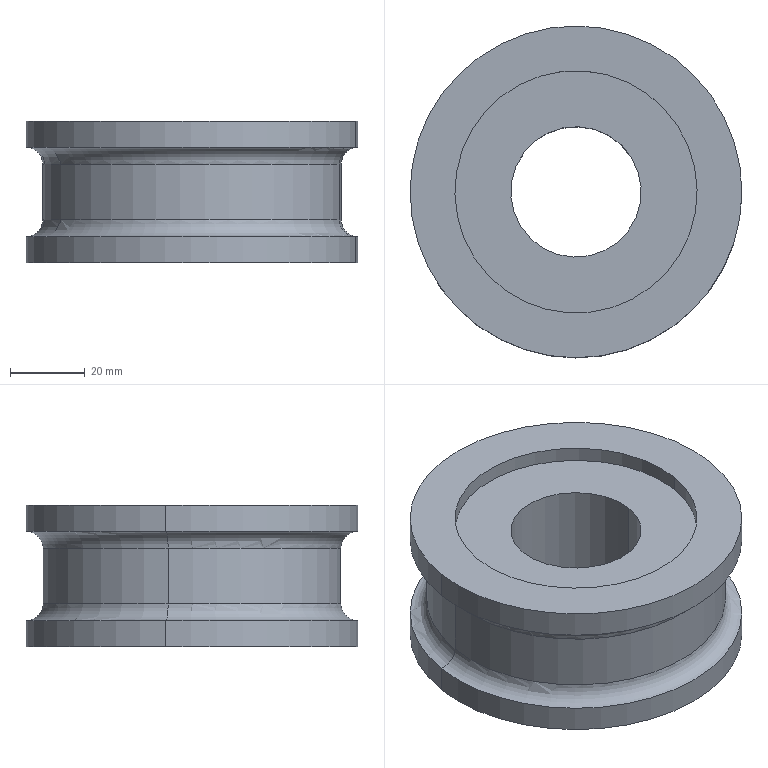Component | SolidWorks | 12AFixedFlatGrooveLargeWheel-EngravingAndMillingAxis-2_12AFlatSlotLargeStraighteningWheel-1 | 1 solid | 20 faces | box 89 x 89 x 38 mm | volume 154563 mm3 | cylinder 12 | torus 4 | plane 4 | commonest cylinder face diameters 65 x4 89 x4 35 x2 80 x2 | material GCr15
build123d program:
from build123d import *


with BuildPart() as part:
    # Sketch1 → Revolve1 (revolve)
    with BuildSketch(Plane.XY, mode=Mode.PRIVATE) as revolve1_sk:
        with BuildLine():
            Line((0, 32.5), (0, 44.5))
            Line((0, 44.5), (7, 44.5))
            ThreePointArc((7, 44.5), (8.318, 41.318), (11.5, 40))
            Line((11.5, 40), (26.5, 40))
            ThreePointArc((26.5, 40), (29.682, 41.318), (31, 44.5))
            Line((31, 44.5), (38, 44.5))
            Line((38, 44.5), (38, 32.5))
            Line((38, 32.5), (34, 32.5))
            Line((34, 32.5), (34, 17.5))
            Line((34, 17.5), (4, 17.5))
            Line((4, 17.5), (4, 32.5))
            Line((4, 32.5), (0, 32.5))
        make_face()
    revolve(revolve1_sk.sketch.rotate(Axis((0, 0, 0), (1, 0, 0)), 180), axis=Axis((0, 0, 0), (1, 0, 0)))


solid = part.part

# Placed as in the assembly
solid = solid.moved(Location((-257.402, 59.038, 55.75), (0, 90, 0)))
STEP:
#1=COLOUR_RGB('',0.7922,0.8196,0.9333);
#2=FILL_AREA_STYLE_COLOUR('',#1);
#3=FILL_AREA_STYLE('',(#2));
#4=SURFACE_STYLE_FILL_AREA(#3);
#5=SURFACE_SIDE_STYLE('',(#4));
#6=SURFACE_STYLE_USAGE(.BOTH.,#5);
#7=PRESENTATION_STYLE_ASSIGNMENT((#6));
#8=CARTESIAN_POINT('',(-9.454,2.214,0.8563));
#9=VERTEX_POINT('',#8);
#10=CARTESIAN_POINT('',(-10.814,2.435,0.8563));
#11=VERTEX_POINT('',#10);
#12=CARTESIAN_POINT('',(-10.134,2.324,0.8563));
#13=DIRECTION('',(0.,-0.,1.));
#14=DIRECTION('',(-0.9871,0.1604,0.));
#15=AXIS2_PLACEMENT_3D('',#12,#13,#14);
#16=CIRCLE('',#15,0.689);
#17=EDGE_CURVE('',#9,#11,#16,.T.);
#18=ORIENTED_EDGE('',*,*,#17,.F.);
#19=CARTESIAN_POINT('',(-9.454,2.214,2.037));
#20=VERTEX_POINT('',#19);
#21=CARTESIAN_POINT('',(-9.454,2.214,2.195));
#22=DIRECTION('',(0.,-0.,1.));
#23=VECTOR('',#22,39.37);
#24=LINE('',#21,#23);
#25=EDGE_CURVE('',#9,#20,#24,.T.);
#26=ORIENTED_EDGE('',*,*,#25,.T.);
#27=CARTESIAN_POINT('',(-10.814,2.435,2.037));
#28=VERTEX_POINT('',#27);
#29=CARTESIAN_POINT('',(-10.134,2.324,2.037));
#30=DIRECTION('',(0.,-0.,1.));
#31=DIRECTION('',(-0.9871,0.1604,0.));
#32=AXIS2_PLACEMENT_3D('',#29,#30,#31);
#33=CIRCLE('',#32,0.689);
#34=EDGE_CURVE('',#20,#28,#33,.T.);
#35=ORIENTED_EDGE('',*,*,#34,.T.);
#36=CARTESIAN_POINT('',(-10.814,2.435,2.195));
#37=DIRECTION('',(0.,-0.,1.));
#38=VECTOR('',#37,39.37);
#39=LINE('',#36,#38);
#40=EDGE_CURVE('',#11,#28,#39,.T.);
#41=ORIENTED_EDGE('',*,*,#40,.F.);
#42=EDGE_LOOP('',(#18,#26,#35,#41));
#43=FACE_OUTER_BOUND('',#42,.T.);
#44=CARTESIAN_POINT('',(-10.134,2.324,2.195));
#45=DIRECTION('',(0.,-0.,1.));
#46=DIRECTION('',(-0.9871,0.1604,0.));
#47=AXIS2_PLACEMENT_3D('',#44,#45,#46);
#48=CYLINDRICAL_SURFACE('',#47,0.689);
#49=ADVANCED_FACE('',(#43),#48,.F.);
#50=CARTESIAN_POINT('',(-8.871,2.119,2.037));
#51=VERTEX_POINT('',#50);
#52=CARTESIAN_POINT('',(-11.397,2.53,2.037));
#53=VERTEX_POINT('',#52);
#54=CARTESIAN_POINT('',(-10.134,2.324,2.037));
#55=DIRECTION('',(0.,-0.,1.));
#56=DIRECTION('',(-0.9871,0.1604,0.));
#57=AXIS2_PLACEMENT_3D('',#54,#55,#56);
#58=CIRCLE('',#57,1.28);
#59=EDGE_CURVE('',#51,#53,#58,.T.);
#60=ORIENTED_EDGE('',*,*,#59,.F.);
#61=CARTESIAN_POINT('',(-8.871,2.119,2.195));
#62=VERTEX_POINT('',#61);
#63=CARTESIAN_POINT('',(-8.871,2.119,2.195));
#64=DIRECTION('',(0.,-0.,1.));
#65=VECTOR('',#64,39.37);
#66=LINE('',#63,#65);
#67=EDGE_CURVE('',#51,#62,#66,.T.);
#68=ORIENTED_EDGE('',*,*,#67,.T.);
#69=CARTESIAN_POINT('',(-11.397,2.53,2.195));
#70=VERTEX_POINT('',#69);
#71=CARTESIAN_POINT('',(-10.134,2.324,2.195));
#72=DIRECTION('',(0.,-0.,1.));
#73=DIRECTION('',(-0.9871,0.1604,0.));
#74=AXIS2_PLACEMENT_3D('',#71,#72,#73);
#75=CIRCLE('',#74,1.28);
#76=EDGE_CURVE('',#62,#70,#75,.T.);
#77=ORIENTED_EDGE('',*,*,#76,.T.);
#78=CARTESIAN_POINT('',(-11.397,2.53,2.195));
#79=DIRECTION('',(0.,-0.,1.));
#80=VECTOR('',#79,39.37);
#81=LINE('',#78,#80);
#82=EDGE_CURVE('',#53,#70,#81,.T.);
#83=ORIENTED_EDGE('',*,*,#82,.F.);
#84=EDGE_LOOP('',(#60,#68,#77,#83));
#85=FACE_OUTER_BOUND('',#84,.T.);
#86=CARTESIAN_POINT('',(-10.134,2.324,2.195));
#87=DIRECTION('',(0.,-0.,1.));
#88=DIRECTION('',(-0.9871,0.1604,0.));
#89=AXIS2_PLACEMENT_3D('',#86,#87,#88);
#90=CYLINDRICAL_SURFACE('',#89,1.28);
#91=ADVANCED_FACE('',(#85),#90,.F.);
#92=CARTESIAN_POINT('',(-11.863,2.605,1.919));
#93=VERTEX_POINT('',#92);
#94=CARTESIAN_POINT('',(-8.405,2.043,1.919));
#95=VERTEX_POINT('',#94);
#96=CARTESIAN_POINT('',(-10.134,2.324,1.919));
#97=DIRECTION('',(0.,-0.,1.));
#98=DIRECTION('',(-0.9871,0.1604,0.));
#99=AXIS2_PLACEMENT_3D('',#96,#97,#98);
#100=CIRCLE('',#99,1.752);
#101=EDGE_CURVE('',#93,#95,#100,.T.);
#102=ORIENTED_EDGE('',*,*,#101,.T.);
#103=CARTESIAN_POINT('',(-8.405,2.043,2.195));
#104=VERTEX_POINT('',#103);
#105=CARTESIAN_POINT('',(-8.405,2.043,2.195));
#106=DIRECTION('',(0.,-0.,1.));
#107=VECTOR('',#106,39.37);
#108=LINE('',#105,#107);
#109=EDGE_CURVE('',#95,#104,#108,.T.);
#110=ORIENTED_EDGE('',*,*,#109,.T.);
#111=CARTESIAN_POINT('',(-11.863,2.605,2.195));
#112=VERTEX_POINT('',#111);
#113=CARTESIAN_POINT('',(-10.134,2.324,2.195));
#114=DIRECTION('',(0.,-0.,1.));
#115=DIRECTION('',(-0.9871,0.1604,0.));
#116=AXIS2_PLACEMENT_3D('',#113,#114,#115);
#117=CIRCLE('',#116,1.752);
#118=EDGE_CURVE('',#112,#104,#117,.T.);
#119=ORIENTED_EDGE('',*,*,#118,.F.);
#120=CARTESIAN_POINT('',(-11.863,2.605,2.195));
#121=DIRECTION('',(0.,-0.,1.));
#122=VECTOR('',#121,39.37);
#123=LINE('',#120,#122);
#124=EDGE_CURVE('',#93,#112,#123,.T.);
#125=ORIENTED_EDGE('',*,*,#124,.F.);
#126=EDGE_LOOP('',(#102,#110,#119,#125));
#127=FACE_OUTER_BOUND('',#126,.T.);
#128=CARTESIAN_POINT('',(-10.134,2.324,2.195));
#129=DIRECTION('',(0.,-0.,1.));
#130=DIRECTION('',(-0.9871,0.1604,0.));
#131=AXIS2_PLACEMENT_3D('',#128,#129,#130);
#132=CYLINDRICAL_SURFACE('',#131,1.752);
#133=ADVANCED_FACE('',(#127),#132,.T.);
#134=CARTESIAN_POINT('',(-10.134,2.324,1.919));
#135=DIRECTION('',(0.,-0.,1.));
#136=DIRECTION('',(-0.9871,0.1604,0.));
#137=AXIS2_PLACEMENT_3D('',#134,#135,#136);
#138=CIRCLE('',#137,1.752);
#139=EDGE_CURVE('',#95,#93,#138,.T.);
#140=ORIENTED_EDGE('',*,*,#139,.F.);
#141=CARTESIAN_POINT('',(-8.58,2.072,1.742));
#142=VERTEX_POINT('',#141);
#143=CARTESIAN_POINT('',(-8.405,2.043,1.742));
#144=DIRECTION('',(-0.1604,-0.9871,-0.));
#145=DIRECTION('',(0.9871,-0.1604,0.));
#146=AXIS2_PLACEMENT_3D('',#143,#144,#145);
#147=CIRCLE('',#146,0.1772);
#148=EDGE_CURVE('',#95,#142,#147,.T.);
#149=ORIENTED_EDGE('',*,*,#148,.T.);
#150=CARTESIAN_POINT('',(-11.688,2.577,1.742));
#151=VERTEX_POINT('',#150);
#152=CARTESIAN_POINT('',(-10.134,2.324,1.742));
#153=DIRECTION('',(0.,-0.,1.));
#154=DIRECTION('',(-0.9871,0.1604,0.));
#155=AXIS2_PLACEMENT_3D('',#152,#153,#154);
#156=CIRCLE('',#155,1.575);
#157=EDGE_CURVE('',#142,#151,#156,.T.);
#158=ORIENTED_EDGE('',*,*,#157,.T.);
#159=CARTESIAN_POINT('',(-11.863,2.605,1.742));
#160=DIRECTION('',(0.1604,0.9871,0.));
#161=DIRECTION('',(-0.9871,0.1604,0.));
#162=AXIS2_PLACEMENT_3D('',#159,#160,#161);
#163=CIRCLE('',#162,0.1772);
#164=EDGE_CURVE('',#93,#151,#163,.T.);
#165=ORIENTED_EDGE('',*,*,#164,.F.);
#166=EDGE_LOOP('',(#140,#149,#158,#165));
#167=FACE_OUTER_BOUND('',#166,.T.);
#168=CARTESIAN_POINT('',(-10.134,2.324,1.742));
#169=DIRECTION('',(0.,-0.,1.));
#170=DIRECTION('',(-0.9871,0.1604,0.));
#171=AXIS2_PLACEMENT_3D('',#168,#169,#170);
#172=TOROIDAL_SURFACE('',#171,1.752,0.1772);
#173=ADVANCED_FACE('',(#167),#172,.F.);
#174=CARTESIAN_POINT('',(-11.688,2.577,1.152));
#175=VERTEX_POINT('',#174);
#176=CARTESIAN_POINT('',(-8.58,2.072,1.152));
#177=VERTEX_POINT('',#176);
#178=CARTESIAN_POINT('',(-10.134,2.324,1.152));
#179=DIRECTION('',(0.,-0.,1.));
#180=DIRECTION('',(-0.9871,0.1604,0.));
#181=AXIS2_PLACEMENT_3D('',#178,#179,#180);
#182=CIRCLE('',#181,1.575);
#183=EDGE_CURVE('',#175,#177,#182,.T.);
#184=ORIENTED_EDGE('',*,*,#183,.T.);
#185=CARTESIAN_POINT('',(-8.58,2.072,2.195));
#186=DIRECTION('',(0.,-0.,1.));
#187=VECTOR('',#186,39.37);
#188=LINE('',#185,#187);
#189=EDGE_CURVE('',#177,#142,#188,.T.);
#190=ORIENTED_EDGE('',*,*,#189,.T.);
#191=CARTESIAN_POINT('',(-10.134,2.324,1.742));
#192=DIRECTION('',(0.,-0.,1.));
#193=DIRECTION('',(-0.9871,0.1604,0.));
#194=AXIS2_PLACEMENT_3D('',#191,#192,#193);
#195=CIRCLE('',#194,1.575);
#196=EDGE_CURVE('',#151,#142,#195,.T.);
#197=ORIENTED_EDGE('',*,*,#196,.F.);
#198=CARTESIAN_POINT('',(-11.688,2.577,2.195));
#199=DIRECTION('',(0.,-0.,1.));
#200=VECTOR('',#199,39.37);
#201=LINE('',#198,#200);
#202=EDGE_CURVE('',#175,#151,#201,.T.);
#203=ORIENTED_EDGE('',*,*,#202,.F.);
#204=EDGE_LOOP('',(#184,#190,#197,#203));
#205=FACE_OUTER_BOUND('',#204,.T.);
#206=CARTESIAN_POINT('',(-10.134,2.324,2.195));
#207=DIRECTION('',(0.,-0.,1.));
#208=DIRECTION('',(-0.9871,0.1604,0.));
#209=AXIS2_PLACEMENT_3D('',#206,#207,#208);
#210=CYLINDRICAL_SURFACE('',#209,1.575);
#211=ADVANCED_FACE('',(#205),#210,.T.);
#212=CARTESIAN_POINT('',(-10.134,2.324,1.152));
#213=DIRECTION('',(0.,-0.,1.));
#214=DIRECTION('',(-0.9871,0.1604,0.));
#215=AXIS2_PLACEMENT_3D('',#212,#213,#214);
#216=CIRCLE('',#215,1.575);
#217=EDGE_CURVE('',#177,#175,#216,.T.);
#218=ORIENTED_EDGE('',*,*,#217,.F.);
#219=CARTESIAN_POINT('',(-8.405,2.043,0.9744));
#220=VERTEX_POINT('',#219);
#221=CARTESIAN_POINT('',(-8.405,2.043,1.152));
#222=DIRECTION('',(-0.1604,-0.9871,-0.));
#223=DIRECTION('',(0.9871,-0.1604,0.));
#224=AXIS2_PLACEMENT_3D('',#221,#222,#223);
#225=CIRCLE('',#224,0.1772);
#226=EDGE_CURVE('',#177,#220,#225,.T.);
#227=ORIENTED_EDGE('',*,*,#226,.T.);
#228=CARTESIAN_POINT('',(-11.863,2.605,0.9744));
#229=VERTEX_POINT('',#228);
#230=CARTESIAN_POINT('',(-10.134,2.324,0.9744));
#231=DIRECTION('',(0.,-0.,1.));
#232=DIRECTION('',(-0.9871,0.1604,0.));
#233=AXIS2_PLACEMENT_3D('',#230,#231,#232);
#234=CIRCLE('',#233,1.752);
#235=EDGE_CURVE('',#220,#229,#234,.T.);
#236=ORIENTED_EDGE('',*,*,#235,.T.);
#237=CARTESIAN_POINT('',(-11.863,2.605,1.152));
#238=DIRECTION('',(0.1604,0.9871,0.));
#239=DIRECTION('',(-0.9871,0.1604,0.));
#240=AXIS2_PLACEMENT_3D('',#237,#238,#239);
#241=CIRCLE('',#240,0.1772);
#242=EDGE_CURVE('',#175,#229,#241,.T.);
#243=ORIENTED_EDGE('',*,*,#242,.F.);
#244=EDGE_LOOP('',(#218,#227,#236,#243));
#245=FACE_OUTER_BOUND('',#244,.T.);
#246=CARTESIAN_POINT('',(-10.134,2.324,1.152));
#247=DIRECTION('',(0.,-0.,1.));
#248=DIRECTION('',(-0.9871,0.1604,0.));
#249=AXIS2_PLACEMENT_3D('',#246,#247,#248);
#250=TOROIDAL_SURFACE('',#249,1.752,0.1772);
#251=ADVANCED_FACE('',(#245),#250,.F.);
#252=CARTESIAN_POINT('',(-11.863,2.605,0.6988));
#253=VERTEX_POINT('',#252);
#254=CARTESIAN_POINT('',(-8.405,2.043,0.6988));
#255=VERTEX_POINT('',#254);
#256=CARTESIAN_POINT('',(-10.134,2.324,0.6988));
#257=DIRECTION('',(0.,-0.,1.));
#258=DIRECTION('',(-0.9871,0.1604,0.));
#259=AXIS2_PLACEMENT_3D('',#256,#257,#258);
#260=CIRCLE('',#259,1.752);
#261=EDGE_CURVE('',#253,#255,#260,.T.);
#262=ORIENTED_EDGE('',*,*,#261,.T.);
#263=CARTESIAN_POINT('',(-8.405,2.043,2.195));
#264=DIRECTION('',(0.,-0.,1.));
#265=VECTOR('',#264,39.37);
#266=LINE('',#263,#265);
#267=EDGE_CURVE('',#255,#220,#266,.T.);
#268=ORIENTED_EDGE('',*,*,#267,.T.);
#269=CARTESIAN_POINT('',(-10.134,2.324,0.9744));
#270=DIRECTION('',(0.,-0.,1.));
#271=DIRECTION('',(-0.9871,0.1604,0.));
#272=AXIS2_PLACEMENT_3D('',#269,#270,#271);
#273=CIRCLE('',#272,1.752);
#274=EDGE_CURVE('',#229,#220,#273,.T.);
#275=ORIENTED_EDGE('',*,*,#274,.F.);
#276=CARTESIAN_POINT('',(-11.863,2.605,2.195));
#277=DIRECTION('',(0.,-0.,1.));
#278=VECTOR('',#277,39.37);
#279=LINE('',#276,#278);
#280=EDGE_CURVE('',#253,#229,#279,.T.);
#281=ORIENTED_EDGE('',*,*,#280,.F.);
#282=EDGE_LOOP('',(#262,#268,#275,#281));
#283=FACE_OUTER_BOUND('',#282,.T.);
#284=CARTESIAN_POINT('',(-10.134,2.324,2.195));
#285=DIRECTION('',(0.,-0.,1.));
#286=DIRECTION('',(-0.9871,0.1604,0.));
#287=AXIS2_PLACEMENT_3D('',#284,#285,#286);
#288=CYLINDRICAL_SURFACE('',#287,1.752);
#289=ADVANCED_FACE('',(#283),#288,.T.);
#290=CARTESIAN_POINT('',(-8.871,2.119,0.6988));
#291=VERTEX_POINT('',#290);
#292=CARTESIAN_POINT('',(-11.397,2.53,0.6988));
#293=VERTEX_POINT('',#292);
#294=CARTESIAN_POINT('',(-10.134,2.324,0.6988));
#295=DIRECTION('',(0.,-0.,1.));
#296=DIRECTION('',(-0.9871,0.1604,0.));
#297=AXIS2_PLACEMENT_3D('',#294,#295,#296);
#298=CIRCLE('',#297,1.28);
#299=EDGE_CURVE('',#291,#293,#298,.T.);
#300=ORIENTED_EDGE('',*,*,#299,.F.);
#301=CARTESIAN_POINT('',(-8.871,2.119,0.8563));
#302=VERTEX_POINT('',#301);
#303=CARTESIAN_POINT('',(-8.871,2.119,2.195));
#304=DIRECTION('',(0.,-0.,1.));
#305=VECTOR('',#304,39.37);
#306=LINE('',#303,#305);
#307=EDGE_CURVE('',#291,#302,#306,.T.);
#308=ORIENTED_EDGE('',*,*,#307,.T.);
#309=CARTESIAN_POINT('',(-11.397,2.53,0.8563));
#310=VERTEX_POINT('',#309);
#311=CARTESIAN_POINT('',(-10.134,2.324,0.8563));
#312=DIRECTION('',(0.,-0.,1.));
#313=DIRECTION('',(-0.9871,0.1604,0.));
#314=AXIS2_PLACEMENT_3D('',#311,#312,#313);
#315=CIRCLE('',#314,1.28);
#316=EDGE_CURVE('',#302,#310,#315,.T.);
#317=ORIENTED_EDGE('',*,*,#316,.T.);
#318=CARTESIAN_POINT('',(-11.397,2.53,2.195));
#319=DIRECTION('',(0.,-0.,1.));
#320=VECTOR('',#319,39.37);
#321=LINE('',#318,#320);
#322=EDGE_CURVE('',#293,#310,#321,.T.);
#323=ORIENTED_EDGE('',*,*,#322,.F.);
#324=EDGE_LOOP('',(#300,#308,#317,#323));
#325=FACE_OUTER_BOUND('',#324,.T.);
#326=CARTESIAN_POINT('',(-10.134,2.324,2.195));
#327=DIRECTION('',(0.,-0.,1.));
#328=DIRECTION('',(-0.9871,0.1604,0.));
#329=AXIS2_PLACEMENT_3D('',#326,#327,#328);
#330=CYLINDRICAL_SURFACE('',#329,1.28);
#331=ADVANCED_FACE('',(#325),#330,.F.);
#332=ORIENTED_EDGE('',*,*,#307,.F.);
#333=CARTESIAN_POINT('',(-10.134,2.324,0.6988));
#334=DIRECTION('',(0.,-0.,1.));
#335=DIRECTION('',(-0.9871,0.1604,0.));
#336=AXIS2_PLACEMENT_3D('',#333,#334,#335);
#337=CIRCLE('',#336,1.28);
#338=EDGE_CURVE('',#293,#291,#337,.T.);
#339=ORIENTED_EDGE('',*,*,#338,.F.);
#340=ORIENTED_EDGE('',*,*,#322,.T.);
#341=CARTESIAN_POINT('',(-10.134,2.324,0.8563));
#342=DIRECTION('',(0.,-0.,1.));
#343=DIRECTION('',(-0.9871,0.1604,0.));
#344=AXIS2_PLACEMENT_3D('',#341,#342,#343);
#345=CIRCLE('',#344,1.28);
#346=EDGE_CURVE('',#310,#302,#345,.T.);
#347=ORIENTED_EDGE('',*,*,#346,.T.);
#348=EDGE_LOOP('',(#332,#339,#340,#347));
#349=FACE_OUTER_BOUND('',#348,.T.);
#350=CARTESIAN_POINT('',(-10.134,2.324,2.195));
#351=DIRECTION('',(0.,-0.,1.));
#352=DIRECTION('',(-0.9871,0.1604,0.));
#353=AXIS2_PLACEMENT_3D('',#350,#351,#352);
#354=CYLINDRICAL_SURFACE('',#353,1.28);
#355=ADVANCED_FACE('',(#349),#354,.F.);
#356=ORIENTED_EDGE('',*,*,#261,.F.);
#357=CARTESIAN_POINT('',(-10.134,2.324,0.6988));
#358=DIRECTION('',(0.,-0.,1.));
#359=DIRECTION('',(-0.9871,0.1604,0.));
#360=AXIS2_PLACEMENT_3D('',#357,#358,#359);
#361=CIRCLE('',#360,1.752);
#362=EDGE_CURVE('',#255,#253,#361,.T.);
#363=ORIENTED_EDGE('',*,*,#362,.F.);
#364=EDGE_LOOP('',(#356,#363));
#365=FACE_OUTER_BOUND('',#364,.T.);
#366=ORIENTED_EDGE('',*,*,#338,.T.);
#367=ORIENTED_EDGE('',*,*,#299,.T.);
#368=EDGE_LOOP('',(#366,#367));
#369=FACE_BOUND('',#368,.T.);
#370=CARTESIAN_POINT('',(-8.405,2.043,0.6988));
#371=DIRECTION('',(0.,-0.,1.));
#372=DIRECTION('',(-0.9871,0.1604,0.));
#373=AXIS2_PLACEMENT_3D('',#370,#371,#372);
#374=PLANE('',#373);
#375=ADVANCED_FACE('',(#365,#369),#374,.F.);
#376=ORIENTED_EDGE('',*,*,#267,.F.);
#377=ORIENTED_EDGE('',*,*,#362,.T.);
#378=ORIENTED_EDGE('',*,*,#280,.T.);
#379=ORIENTED_EDGE('',*,*,#235,.F.);
#380=EDGE_LOOP('',(#376,#377,#378,#379));
#381=FACE_OUTER_BOUND('',#380,.T.);
#382=CARTESIAN_POINT('',(-10.134,2.324,2.195));
#383=DIRECTION('',(0.,-0.,1.));
#384=DIRECTION('',(-0.9871,0.1604,0.));
#385=AXIS2_PLACEMENT_3D('',#382,#383,#384);
#386=CYLINDRICAL_SURFACE('',#385,1.752);
#387=ADVANCED_FACE('',(#381),#386,.T.);
#388=ORIENTED_EDGE('',*,*,#226,.F.);
#389=ORIENTED_EDGE('',*,*,#183,.F.);
#390=ORIENTED_EDGE('',*,*,#242,.T.);
#391=ORIENTED_EDGE('',*,*,#274,.T.);
#392=EDGE_LOOP('',(#388,#389,#390,#391));
#393=FACE_OUTER_BOUND('',#392,.T.);
#394=CARTESIAN_POINT('',(-10.134,2.324,1.152));
#395=DIRECTION('',(0.,-0.,1.));
#396=DIRECTION('',(-0.9871,0.1604,0.));
#397=AXIS2_PLACEMENT_3D('',#394,#395,#396);
#398=TOROIDAL_SURFACE('',#397,1.752,0.1772);
#399=ADVANCED_FACE('',(#393),#398,.F.);
#400=ORIENTED_EDGE('',*,*,#189,.F.);
#401=ORIENTED_EDGE('',*,*,#217,.T.);
#402=ORIENTED_EDGE('',*,*,#202,.T.);
#403=ORIENTED_EDGE('',*,*,#157,.F.);
#404=EDGE_LOOP('',(#400,#401,#402,#403));
#405=FACE_OUTER_BOUND('',#404,.T.);
#406=CARTESIAN_POINT('',(-10.134,2.324,2.195));
#407=DIRECTION('',(0.,-0.,1.));
#408=DIRECTION('',(-0.9871,0.1604,0.));
#409=AXIS2_PLACEMENT_3D('',#406,#407,#408);
#410=CYLINDRICAL_SURFACE('',#409,1.575);
#411=ADVANCED_FACE('',(#405),#410,.T.);
#412=ORIENTED_EDGE('',*,*,#148,.F.);
#413=ORIENTED_EDGE('',*,*,#101,.F.);
#414=ORIENTED_EDGE('',*,*,#164,.T.);
#415=ORIENTED_EDGE('',*,*,#196,.T.);
#416=EDGE_LOOP('',(#412,#413,#414,#415));
#417=FACE_OUTER_BOUND('',#416,.T.);
#418=CARTESIAN_POINT('',(-10.134,2.324,1.742));
#419=DIRECTION('',(0.,-0.,1.));
#420=DIRECTION('',(-0.9871,0.1604,0.));
#421=AXIS2_PLACEMENT_3D('',#418,#419,#420);
#422=TOROIDAL_SURFACE('',#421,1.752,0.1772);
#423=ADVANCED_FACE('',(#417),#422,.F.);
#424=ORIENTED_EDGE('',*,*,#109,.F.);
#425=ORIENTED_EDGE('',*,*,#139,.T.);
#426=ORIENTED_EDGE('',*,*,#124,.T.);
#427=CARTESIAN_POINT('',(-10.134,2.324,2.195));
#428=DIRECTION('',(0.,-0.,1.));
#429=DIRECTION('',(-0.9871,0.1604,0.));
#430=AXIS2_PLACEMENT_3D('',#427,#428,#429);
#431=CIRCLE('',#430,1.752);
#432=EDGE_CURVE('',#104,#112,#431,.T.);
#433=ORIENTED_EDGE('',*,*,#432,.F.);
#434=EDGE_LOOP('',(#424,#425,#426,#433));
#435=FACE_OUTER_BOUND('',#434,.T.);
#436=CARTESIAN_POINT('',(-10.134,2.324,2.195));
#437=DIRECTION('',(0.,-0.,1.));
#438=DIRECTION('',(-0.9871,0.1604,0.));
#439=AXIS2_PLACEMENT_3D('',#436,#437,#438);
#440=CYLINDRICAL_SURFACE('',#439,1.752);
#441=ADVANCED_FACE('',(#435),#440,.T.);
#442=CARTESIAN_POINT('',(-10.134,2.324,2.195));
#443=DIRECTION('',(0.,-0.,1.));
#444=DIRECTION('',(-0.9871,0.1604,0.));
#445=AXIS2_PLACEMENT_3D('',#442,#443,#444);
#446=CIRCLE('',#445,1.28);
#447=EDGE_CURVE('',#70,#62,#446,.T.);
#448=ORIENTED_EDGE('',*,*,#447,.F.);
#449=ORIENTED_EDGE('',*,*,#76,.F.);
#450=EDGE_LOOP('',(#448,#449));
#451=FACE_BOUND('',#450,.T.);
#452=ORIENTED_EDGE('',*,*,#118,.T.);
#453=ORIENTED_EDGE('',*,*,#432,.T.);
#454=EDGE_LOOP('',(#452,#453));
#455=FACE_OUTER_BOUND('',#454,.T.);
#456=CARTESIAN_POINT('',(-8.871,2.119,2.195));
#457=DIRECTION('',(-0.,0.,-1.));
#458=DIRECTION('',(0.9871,-0.1604,-0.));
#459=AXIS2_PLACEMENT_3D('',#456,#457,#458);
#460=PLANE('',#459);
#461=ADVANCED_FACE('',(#451,#455),#460,.F.);
#462=ORIENTED_EDGE('',*,*,#67,.F.);
#463=CARTESIAN_POINT('',(-10.134,2.324,2.037));
#464=DIRECTION('',(0.,-0.,1.));
#465=DIRECTION('',(-0.9871,0.1604,0.));
#466=AXIS2_PLACEMENT_3D('',#463,#464,#465);
#467=CIRCLE('',#466,1.28);
#468=EDGE_CURVE('',#53,#51,#467,.T.);
#469=ORIENTED_EDGE('',*,*,#468,.F.);
#470=ORIENTED_EDGE('',*,*,#82,.T.);
#471=ORIENTED_EDGE('',*,*,#447,.T.);
#472=EDGE_LOOP('',(#462,#469,#470,#471));
#473=FACE_OUTER_BOUND('',#472,.T.);
#474=CARTESIAN_POINT('',(-10.134,2.324,2.195));
#475=DIRECTION('',(0.,-0.,1.));
#476=DIRECTION('',(-0.9871,0.1604,0.));
#477=AXIS2_PLACEMENT_3D('',#474,#475,#476);
#478=CYLINDRICAL_SURFACE('',#477,1.28);
#479=ADVANCED_FACE('',(#473),#478,.F.);
#480=CARTESIAN_POINT('',(-10.134,2.324,2.037));
#481=DIRECTION('',(0.,-0.,1.));
#482=DIRECTION('',(-0.9871,0.1604,0.));
#483=AXIS2_PLACEMENT_3D('',#480,#481,#482);
#484=CIRCLE('',#483,0.689);
#485=EDGE_CURVE('',#28,#20,#484,.T.);
#486=ORIENTED_EDGE('',*,*,#485,.F.);
#487=ORIENTED_EDGE('',*,*,#34,.F.);
#488=EDGE_LOOP('',(#486,#487));
#489=FACE_BOUND('',#488,.T.);
#490=ORIENTED_EDGE('',*,*,#468,.T.);
#491=ORIENTED_EDGE('',*,*,#59,.T.);
#492=EDGE_LOOP('',(#490,#491));
#493=FACE_OUTER_BOUND('',#492,.T.);
#494=CARTESIAN_POINT('',(-8.871,2.119,2.037));
#495=DIRECTION('',(-0.,0.,-1.));
#496=DIRECTION('',(0.9871,-0.1604,-0.));
#497=AXIS2_PLACEMENT_3D('',#494,#495,#496);
#498=PLANE('',#497);
#499=ADVANCED_FACE('',(#489,#493),#498,.F.);
#500=ORIENTED_EDGE('',*,*,#25,.F.);
#501=CARTESIAN_POINT('',(-10.134,2.324,0.8563));
#502=DIRECTION('',(0.,-0.,1.));
#503=DIRECTION('',(-0.9871,0.1604,0.));
#504=AXIS2_PLACEMENT_3D('',#501,#502,#503);
#505=CIRCLE('',#504,0.689);
#506=EDGE_CURVE('',#11,#9,#505,.T.);
#507=ORIENTED_EDGE('',*,*,#506,.F.);
#508=ORIENTED_EDGE('',*,*,#40,.T.);
#509=ORIENTED_EDGE('',*,*,#485,.T.);
#510=EDGE_LOOP('',(#500,#507,#508,#509));
#511=FACE_OUTER_BOUND('',#510,.T.);
#512=CARTESIAN_POINT('',(-10.134,2.324,2.195));
#513=DIRECTION('',(0.,-0.,1.));
#514=DIRECTION('',(-0.9871,0.1604,0.));
#515=AXIS2_PLACEMENT_3D('',#512,#513,#514);
#516=CYLINDRICAL_SURFACE('',#515,0.689);
#517=ADVANCED_FACE('',(#511),#516,.F.);
#518=ORIENTED_EDGE('',*,*,#346,.F.);
#519=ORIENTED_EDGE('',*,*,#316,.F.);
#520=EDGE_LOOP('',(#518,#519));
#521=FACE_OUTER_BOUND('',#520,.T.);
#522=ORIENTED_EDGE('',*,*,#506,.T.);
#523=ORIENTED_EDGE('',*,*,#17,.T.);
#524=EDGE_LOOP('',(#522,#523));
#525=FACE_BOUND('',#524,.T.);
#526=CARTESIAN_POINT('',(-8.871,2.119,0.8563));
#527=DIRECTION('',(0.,-0.,1.));
#528=DIRECTION('',(-0.9871,0.1604,0.));
#529=AXIS2_PLACEMENT_3D('',#526,#527,#528);
#530=PLANE('',#529);
#531=ADVANCED_FACE('',(#521,#525),#530,.F.);
#532=CLOSED_SHELL('',(#49,#91,#133,#173,#211,#251,#289,#331,#355,#375,#387,#399,#411,#423,#441,#461,#479,#499,#517,#531));
#533=MANIFOLD_SOLID_BREP('',#532);
#534=STYLED_ITEM('',(#7),#533);
#535=PRESENTATION_LAYER_ASSIGNMENT('','',(#534));
#536=CARTESIAN_POINT('',(0.,0.,0.));
#537=DIRECTION('',(0.,0.,1.));
#538=DIRECTION('',(1.,0.,0.));
#539=AXIS2_PLACEMENT_3D('',#536,#537,#538);
#540=(LENGTH_UNIT()NAMED_UNIT(*)SI_UNIT($,.METRE.));
#541=LENGTH_MEASURE_WITH_UNIT(LENGTH_MEASURE(0.0254),#540);
#542=DIMENSIONAL_EXPONENTS(1.,0.,0.,0.,0.,0.,0.);
#543=(CONVERSION_BASED_UNIT('',#541)LENGTH_UNIT()NAMED_UNIT(#542));
#544=UNCERTAINTY_MEASURE_WITH_UNIT(LENGTH_MEASURE(0.00001),#543,'','');
#545=(NAMED_UNIT(*)PLANE_ANGLE_UNIT()SI_UNIT($,.RADIAN.));
#546=(NAMED_UNIT(*)SI_UNIT($,.STERADIAN.)SOLID_ANGLE_UNIT());
#547=(GEOMETRIC_REPRESENTATION_CONTEXT(3)GLOBAL_UNCERTAINTY_ASSIGNED_CONTEXT((#544))GLOBAL_UNIT_ASSIGNED_CONTEXT((#543,#545,#546))REPRESENTATION_CONTEXT('',''));
#548=ADVANCED_BREP_SHAPE_REPRESENTATION('',(#533,#539),#547);
#549=(LENGTH_UNIT()NAMED_UNIT(*)SI_UNIT($,.METRE.));
#550=LENGTH_MEASURE_WITH_UNIT(LENGTH_MEASURE(0.0254),#549);
#551=DIMENSIONAL_EXPONENTS(1.,0.,0.,0.,0.,0.,0.);
#552=(CONVERSION_BASED_UNIT('',#550)LENGTH_UNIT()NAMED_UNIT(#551));
#553=UNCERTAINTY_MEASURE_WITH_UNIT(LENGTH_MEASURE(0.00001),#552,'','');
#554=(NAMED_UNIT(*)PLANE_ANGLE_UNIT()SI_UNIT($,.RADIAN.));
#555=(NAMED_UNIT(*)SI_UNIT($,.STERADIAN.)SOLID_ANGLE_UNIT());
#556=(GEOMETRIC_REPRESENTATION_CONTEXT(3)GLOBAL_UNCERTAINTY_ASSIGNED_CONTEXT((#553))GLOBAL_UNIT_ASSIGNED_CONTEXT((#552,#554,#555))REPRESENTATION_CONTEXT('',''));
#557=MECHANICAL_DESIGN_GEOMETRIC_PRESENTATION_REPRESENTATION('',(#534),#556);